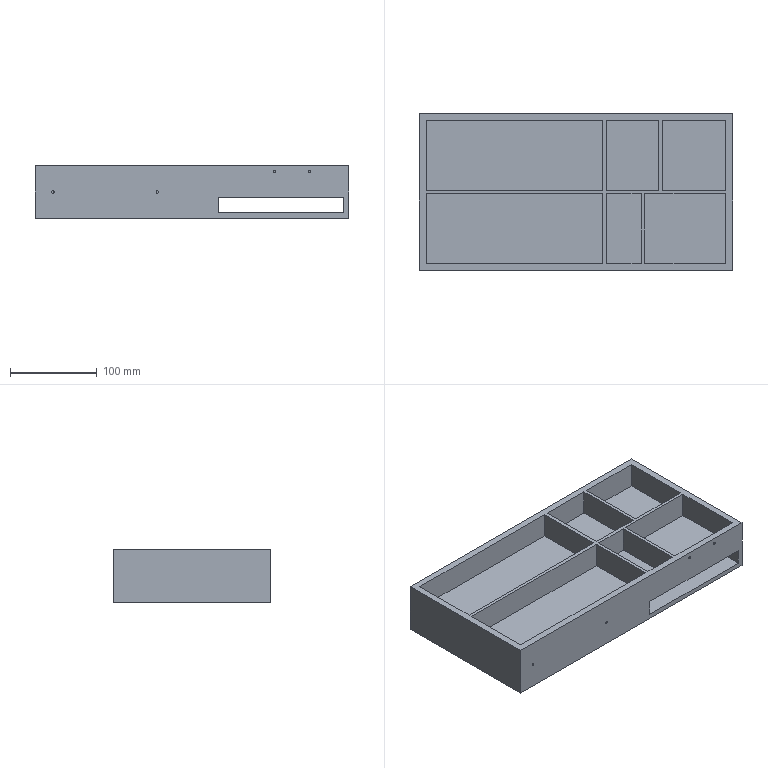Component | NX | INNER_BOX | 1 solid | 60 faces | volume 1806637 mm3 | plane 50 | cylinder 10 | commonest cylinder face diameters 2.8 x8 16 x2